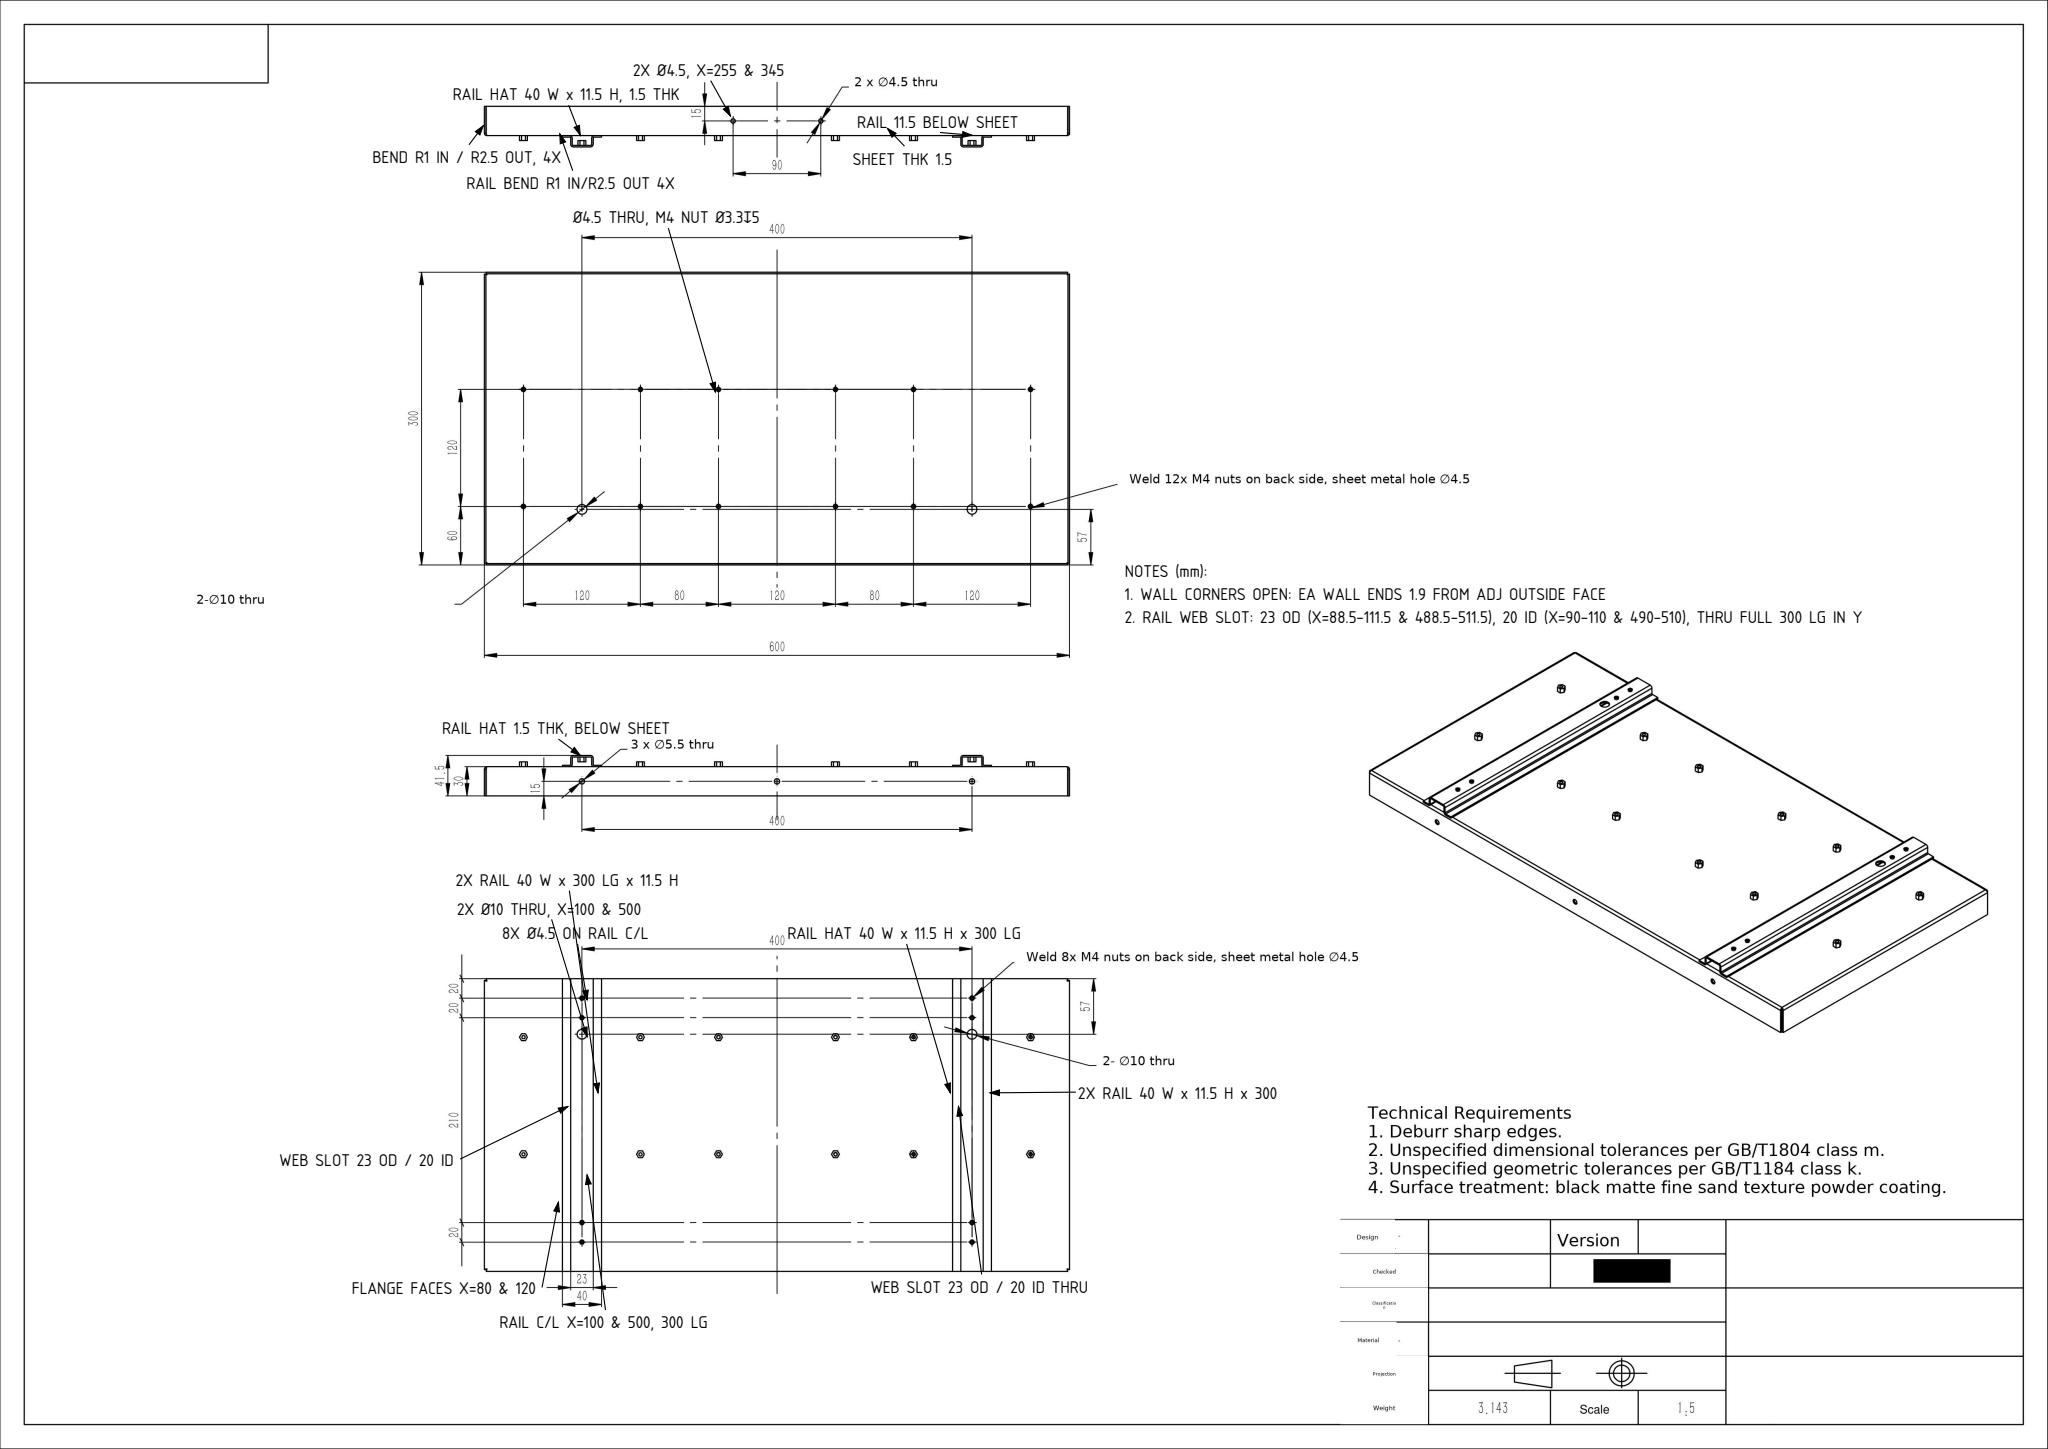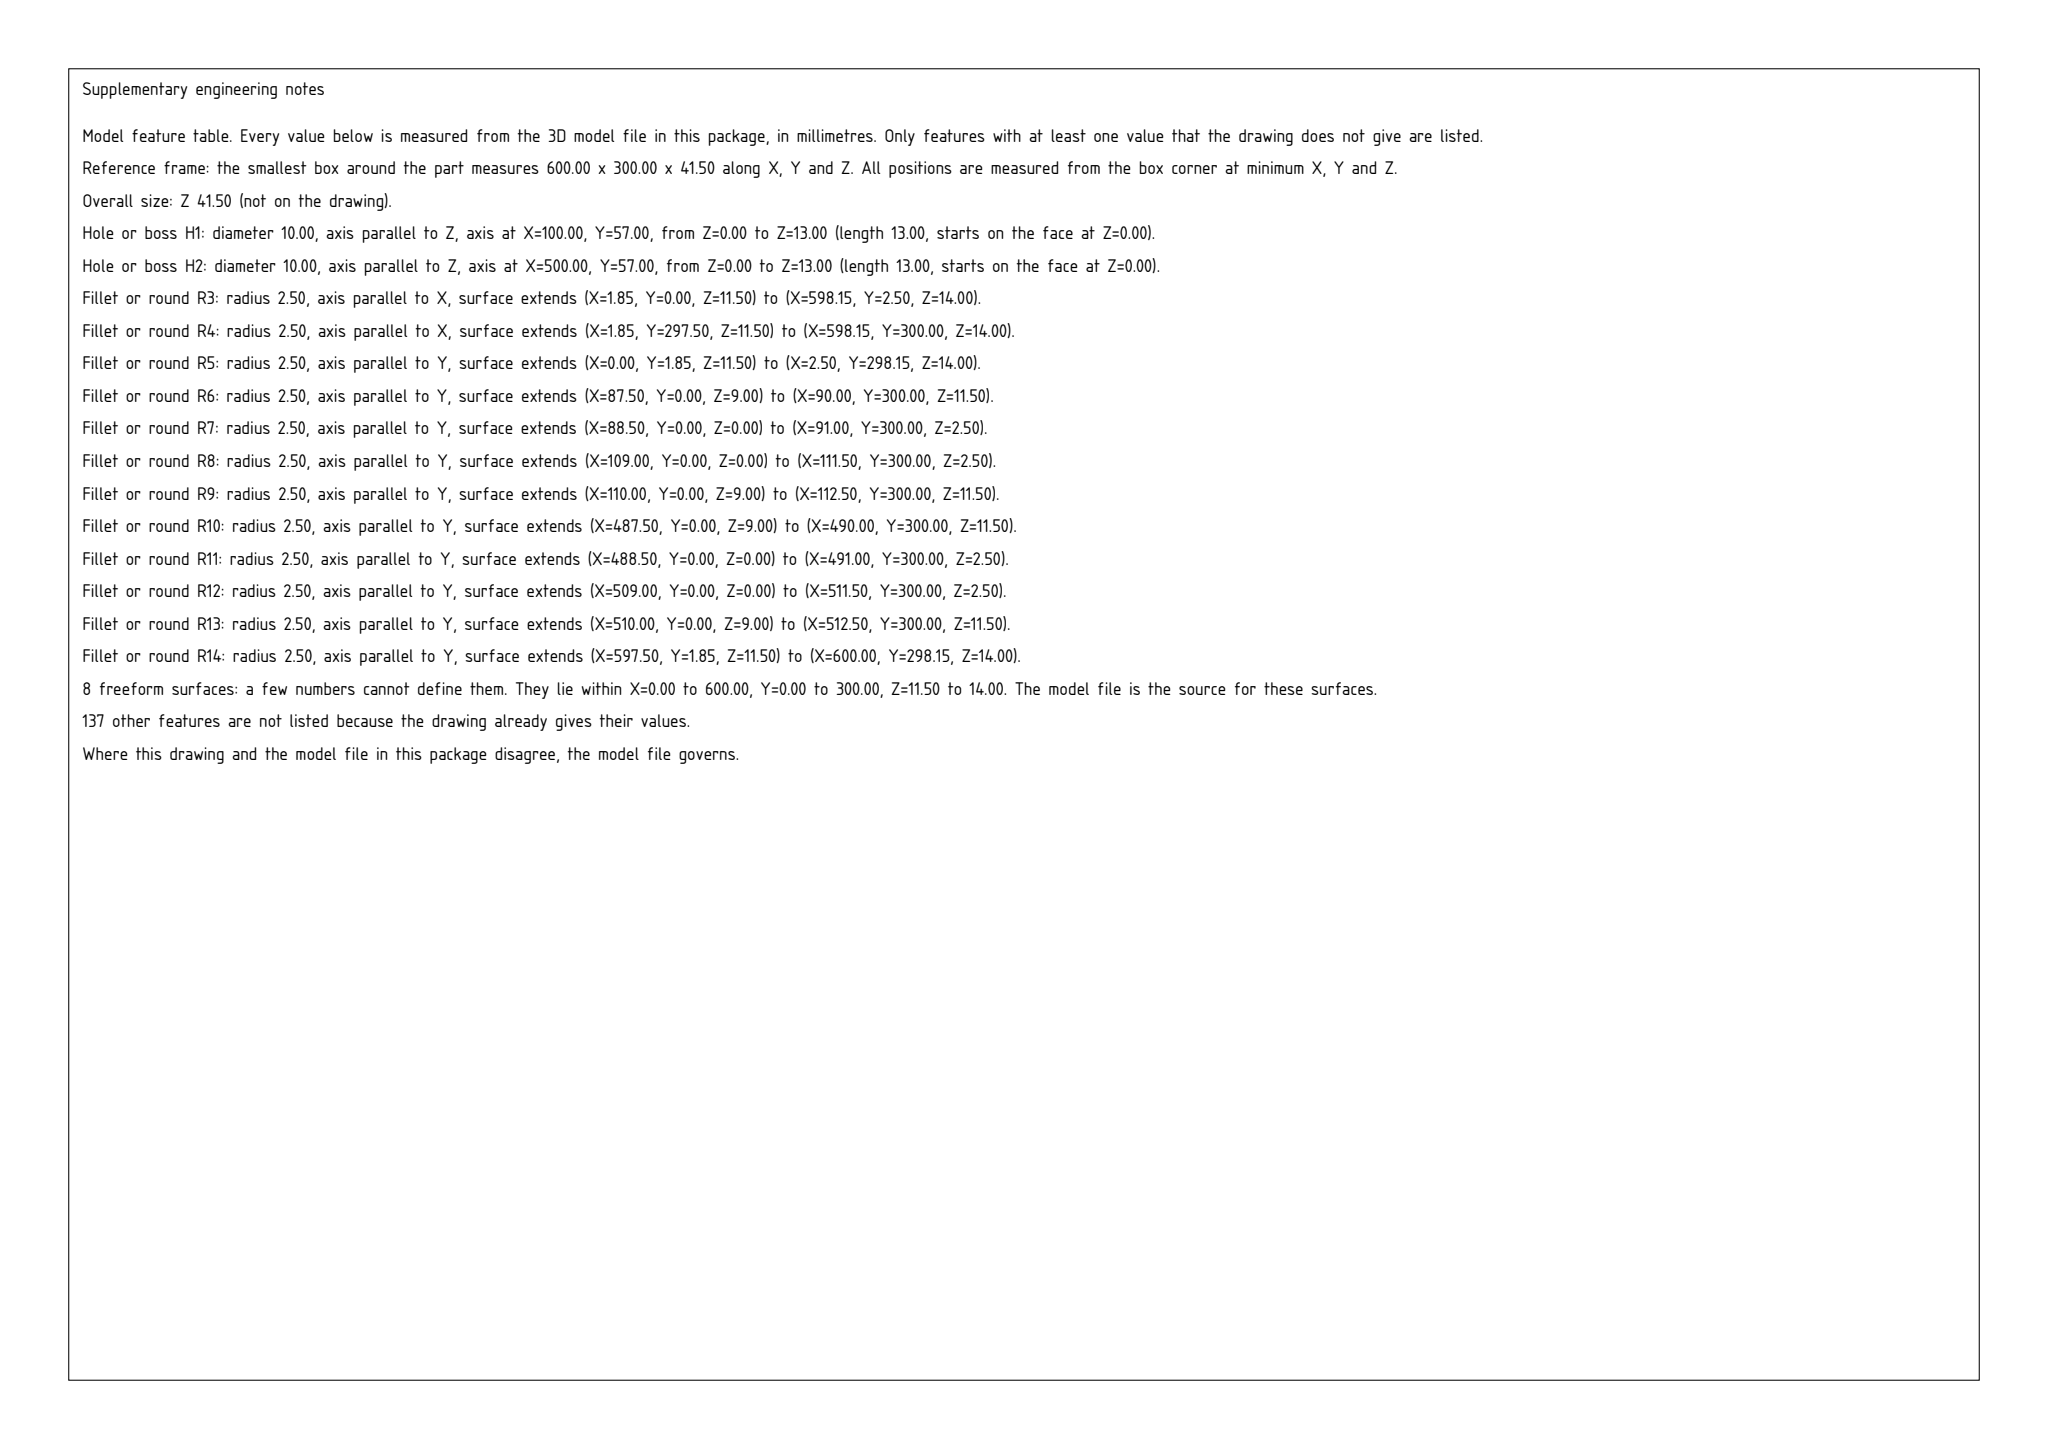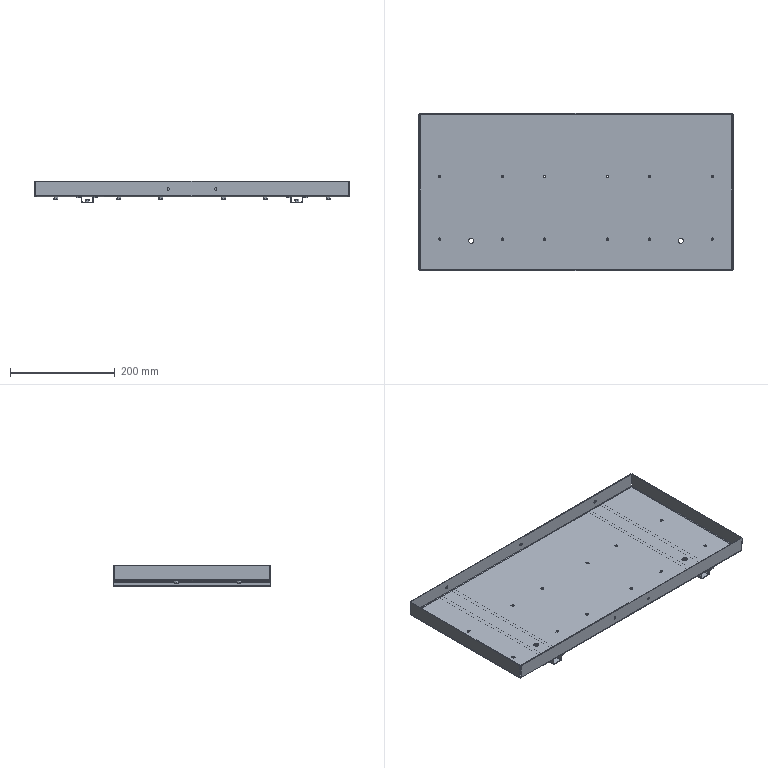Part | SolidWorks | mm | 1 solid | 348 faces | box 600 x 300 x 41.5 mm | volume 397857 mm3 | plane 218 | cylinder 122 | spline 8 | commonest cylinder face diameters 4.5 x44 3.3 x40 2 x12 5 x12 10 x8 5.5 x6
Drawing notes:
BASE SHEET THK 1.5 | from the solid: z planes 0.0 and 1.5; Ø4.5 sheet holes length 1.5
M4 WELD NUT ON BACK: SHEET HOLE Ø4.5 THRU, NUT BORE Ø3.3 x 5 DP TYP | from the solid: Ø4.5 z-holes len 1.5 paired with Ø3.3 z-holes len 5.0 at same x,y
8X Ø4.5 ON RAIL CL X=100 & 500, AT Y=20, 40, 250, 270 | from the solid: Ø4.5/Ø3.3 at x=100.02 & 500.02, y=20.02, 40.02, 250.02, 270.02
2X Ø10 THRU AT X=100 & 500, Y=57 FROM FRONT EDGE | from the solid: [10.0,'z',[100.02,57.02],1.5] and [10.0,'z',[500.02,57.02],1.5]
ALL BENDS 1.5 THK SHEET: R1 INSIDE, R2.5 OUTSIDE (4 WALLS) | from the solid: Bend cylinders dia 2.0 (R1 inside) coaxial with dia 5.0 (R2.5 outside) at x=2.52, x=597.52, y=2.52, y=297.52, all axes at z=14.0; sheet faces 1.5 apart (z=11.5/13.0)
WALL CORNERS OPEN: EA WALL ENDS 1.9 FROM ADJ OUTSIDE FACE | from the solid: Wall faces run y=1.9 to 298.2 and x=1.9 to 598.2 (planes x=0/1.5/598.5/600 extent y [1.9,298.2]; planes y=0/1.5 extent x [1.9,598.2]); small end faces at x=1.9 and 598.2, y=1.9 and 298.2
RAIL SECT: 1.5 THK HAT, 40 W x 11.5 H, WEBS 23 OD / 20 ID, 6.5 DP | from the solid: Rail web/slot faces x=88.5, 90, 110, 111.5 (and 488.5, 490, 510, 511.5) all have z extent [2.5, 9.0] (area 1950 = 300 x 6.5), so web/slot depth is 6.5, not 8.5
2X RAIL 40 W x 300 LG x 11.5 H (NOT 40 H), C/L AT 100 & 500 | from the solid: Rail blocks x 80.02-120.02 and 480.02-520.02, y 0-300 (300 LG), z 0.0-11.5; symmetric about x=100.02 / 500.02
RAILS BELOW BASE: FLANGE TOP TO SHEET UNDERSIDE, 11.5 DOWN | from the solid: Base sheet z=11.5 (bottom) to 13.0 (top); rail z=0.0 to 11.5; overall 41.5 = 30 wall above sheet bottom + 11.5 rail
RAIL HAT BENDS R1 INSIDE / R2.5 OUTSIDE, 4 PLCS EA RAIL | from the solid: Dia2 (R1) & dia5 (R2.5) cyls at x87.52/112.52 z9.0 and x91.02/109.02 z2.5 (and 487.52/512.52, 491.02/509.02)
2X RAIL: HAT SECTION 40 W (X=80-120 & 480-520) x 11.5 H x 300 LG (FULL DEPTH Y=0 TO 300), MOUNTED BELOW BASE SHEET - FLANGE TOP AT SHEET UNDERSIDE Z=11.5, RAIL BOTTOM AT Z=0; C/L AT X=100 & 500 | from the solid: axis_planes x 80.02/120.02 and 480.02/520.02 (40 W, CL 100 & 500); z planes 0.0 (rail bottom) and 11.5 (flange top = sheet underside, sheet top z=13.0, 1.5 THK)
RAIL WEB/SLOT: OD 23 (X=88.5-111.5 & 488.5-511.5), ID 20 (X=90-110 & 490-510), RUNS FULL 300 LG IN Y | from the solid: axis_planes x 88.52, 90.02, 110.02, 111.52, 488.52, 490.02, 510.02, 511.52; y-axis bend cylinders length 300 at x=87.52/91.02/109.02/112.52 and 487.52/491.02/509.02/512.52
2X RAIL: 1.5 THK HAT SECT, 40 W x 11.5 H, FORMED BELOW SHEET UNDERSIDE (HAT TOP AT PART BOTTOM, 11.5 DOWN FROM SHEET UNDERSIDE); NO RAIL ABOVE BASE | from the solid: axis_planes z=0.0 (part bottom) and z=11.5 (sheet underside, count 25); rail bend-radius cylinders dia 2.0/5.0 axis y at z=2.5 and z=9.0
RAIL C/L AT X=100 & 500 FROM LEFT EDGE, FULL 300 LG (RUNS EDGE TO EDGE IN Y); FLANGE OUTSIDE FACES X=80 & 120 AND X=480 & 520 (40 W), WEB SLOT 23 OD / 20 ID | from the solid: cylinders dia 2.0/5.0 axis y at x=87.52, 91.02, 109.02, 112.52 and 487.52, 491.02, 509.02, 512.52, length 300.0; axis_planes x=80.02, 88.52, 90.02, 110.02, 111.52, 120.02 and x=480.02, 488.52, 490.02, 510.02, 511.52, 520.02
2X RAIL: 1.5 THK HAT SECTION 40 W x 11.5 H, BELOW SHEET - FLANGE TOP AT SHEET UNDERSIDE Z=11.5, HAT TOP (PART BOTTOM) AT Z=0; FLANGE OUTSIDE FACES X=80 & 120 AND X=480 & 520, C/L X=100 & 500 FROM LEFT EDGE; NO RAIL ABOVE BASE | from the solid: x planes 80.02/120.02 and 480.02/520.02; z planes 0.0 and 11.5; bbox z 41.5
RAIL WEB SLOT: 23 OD (X=88.5-111.5 & 488.5-511.5), 20 ID (X=90-110 & 490-510), RUNS FULL 300 LG IN Y (Y=0 TO 300) | from the solid: x planes 88.52/111.52, 90.02/110.02, 488.52/511.52, 490.02/510.02; rail cylinders axis y length 300.0 at x=87.52/91.02/109.02/112.52 & 487.52/491.02/509.02/512.52
2X RAIL: HAT SECTION 40 W x 11.5 H x 300 LG, BELOW SHEET ONLY (NO RAIL ABOVE BASE); FLANGE OUTSIDE FACES X=80 & 120 AND X=480 & 520 FROM LEFT EDGE (C/L X=100 & 500); FLANGE TOP AT SHEET UNDERSIDE Z=11.5, HAT TOP AT PART BOTTOM Z=0; RUNS FULL 300 IN Y (Y=0 TO 300) | from the solid: axis_planes x=80.02/120.02 and 480.02/520.02; z planes 0.0 and 11.5; y-axis cylinders at x=87.52/112.52/487.52/512.52 length 300.0; bbox_xyz 600.03 x 300.03 x 41.5
RAIL WEB SLOT: 23 OD (X=88.5-111.5 & 488.5-511.5), 20 ID (X=90-110 & 490-510), THRU FULL 300 LG IN Y | from the solid: axis_planes x=88.52, 90.02, 110.02, 111.52, 488.52, 490.02, 510.02, 511.52; y-axis cylinders at those x, length 300.0
WALL HOLES (FRONT LONG WALL, 1.5 THK): 2X Ø4.5 THRU AT X=255 & 345 FROM LEFT EDGE (SYM ABOUT 600 C/L, 90 APART), AXIS PERP WALL, HOLE C/L Z=26.5 ABOVE PART BOTTOM | from the solid: cylinders: hole/bore Ø4.5 axis y at [255.0, null, 26.5] and [345.0, null, 26.5], from y=0.0 to y=1.5 (1.5 thk wall)